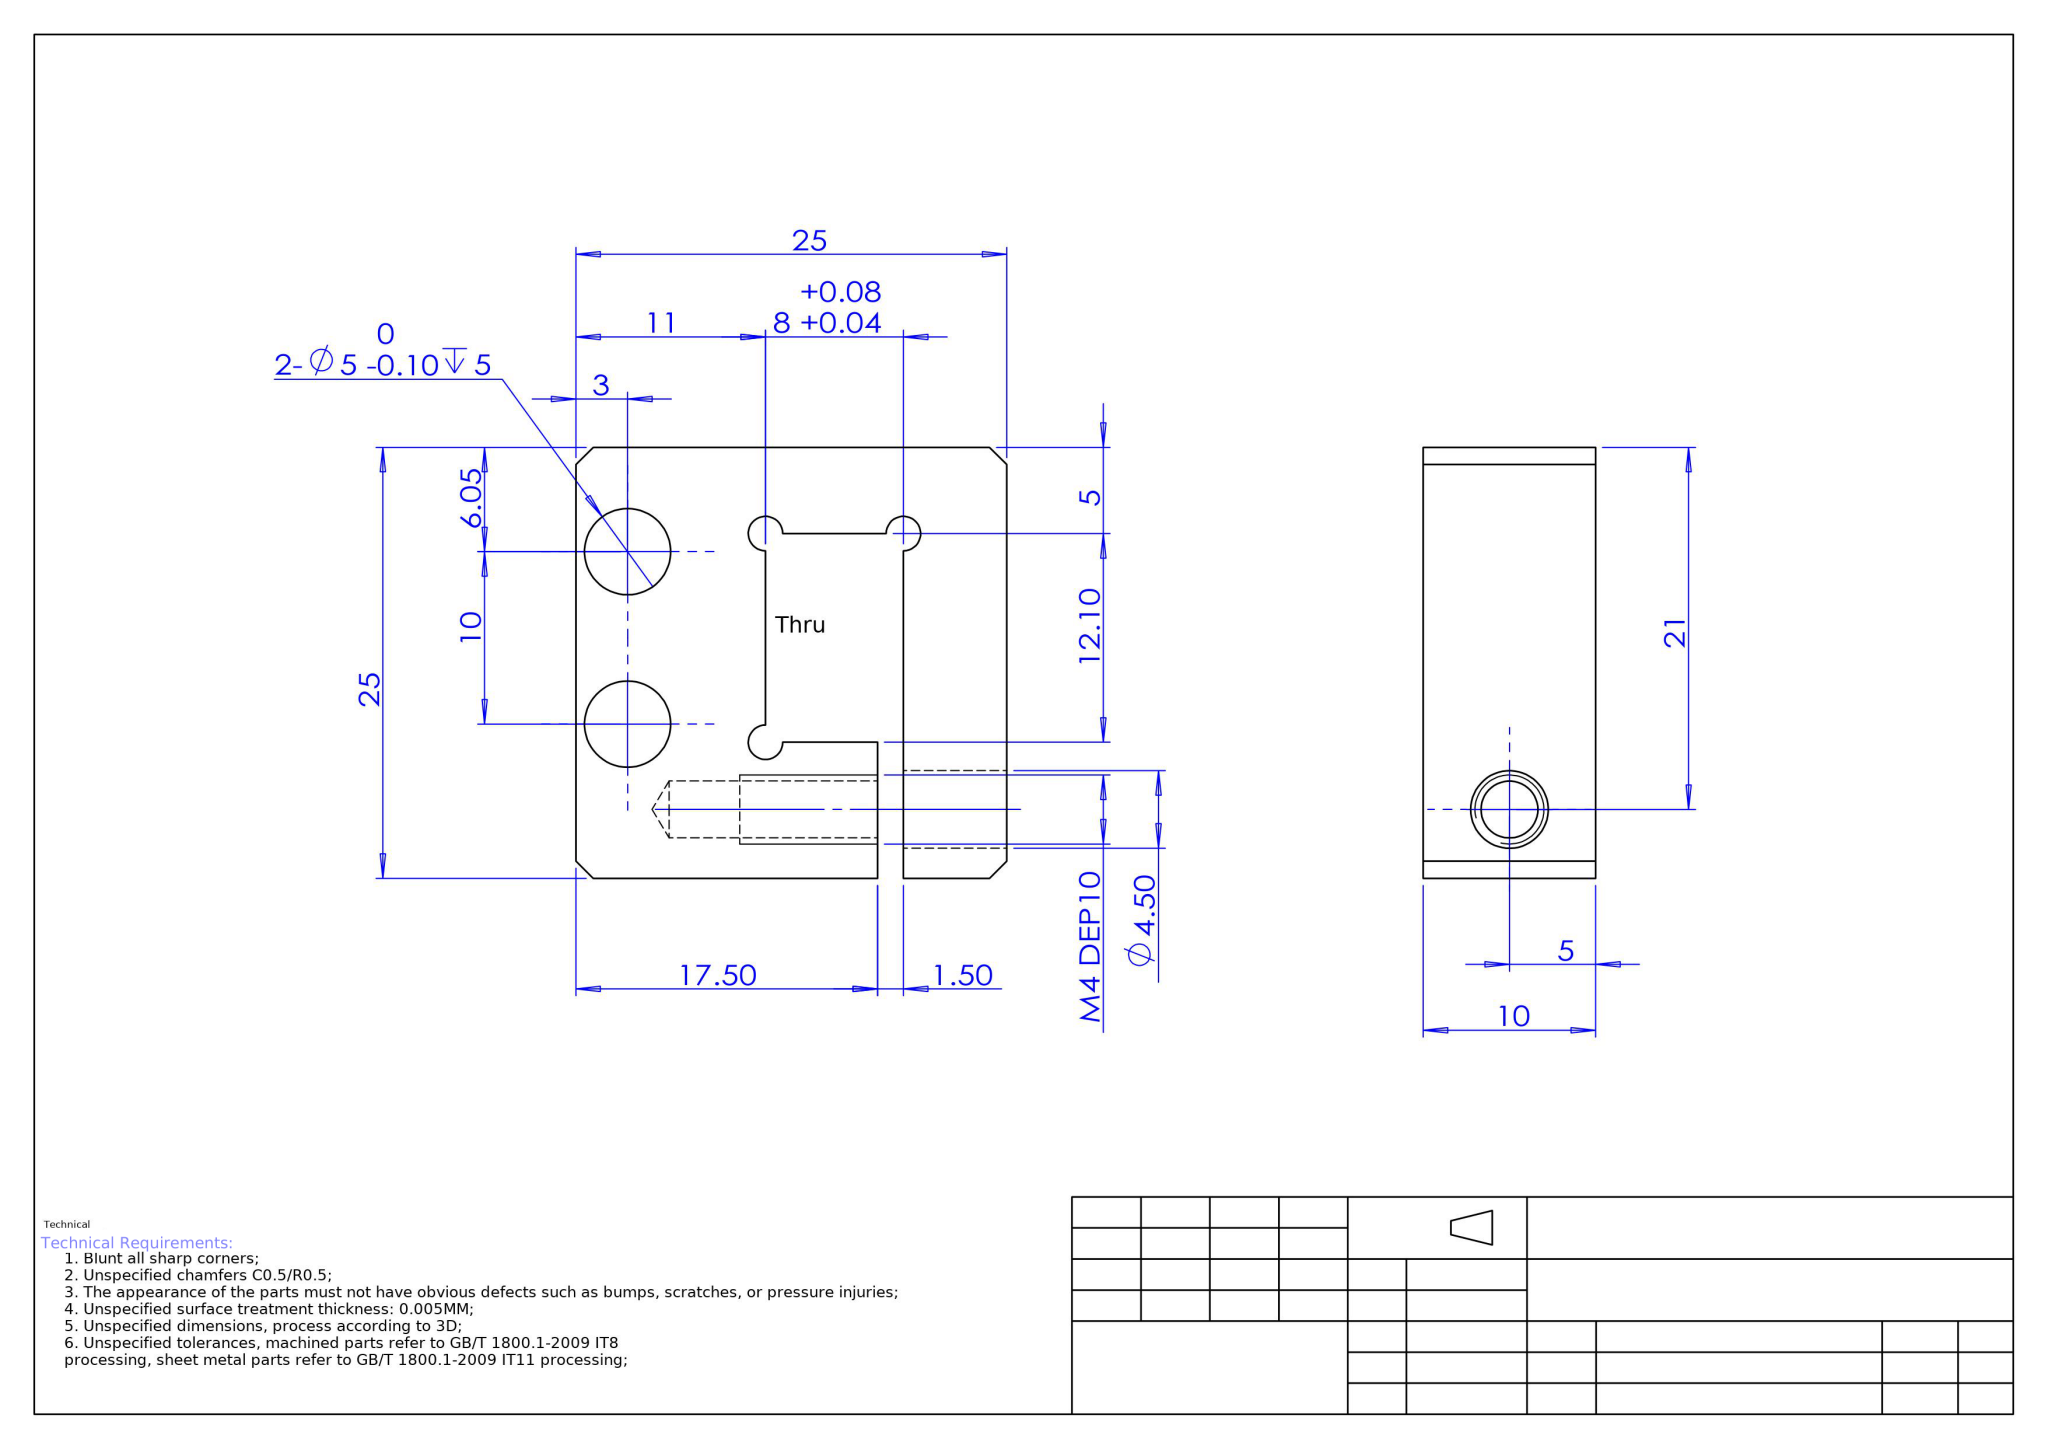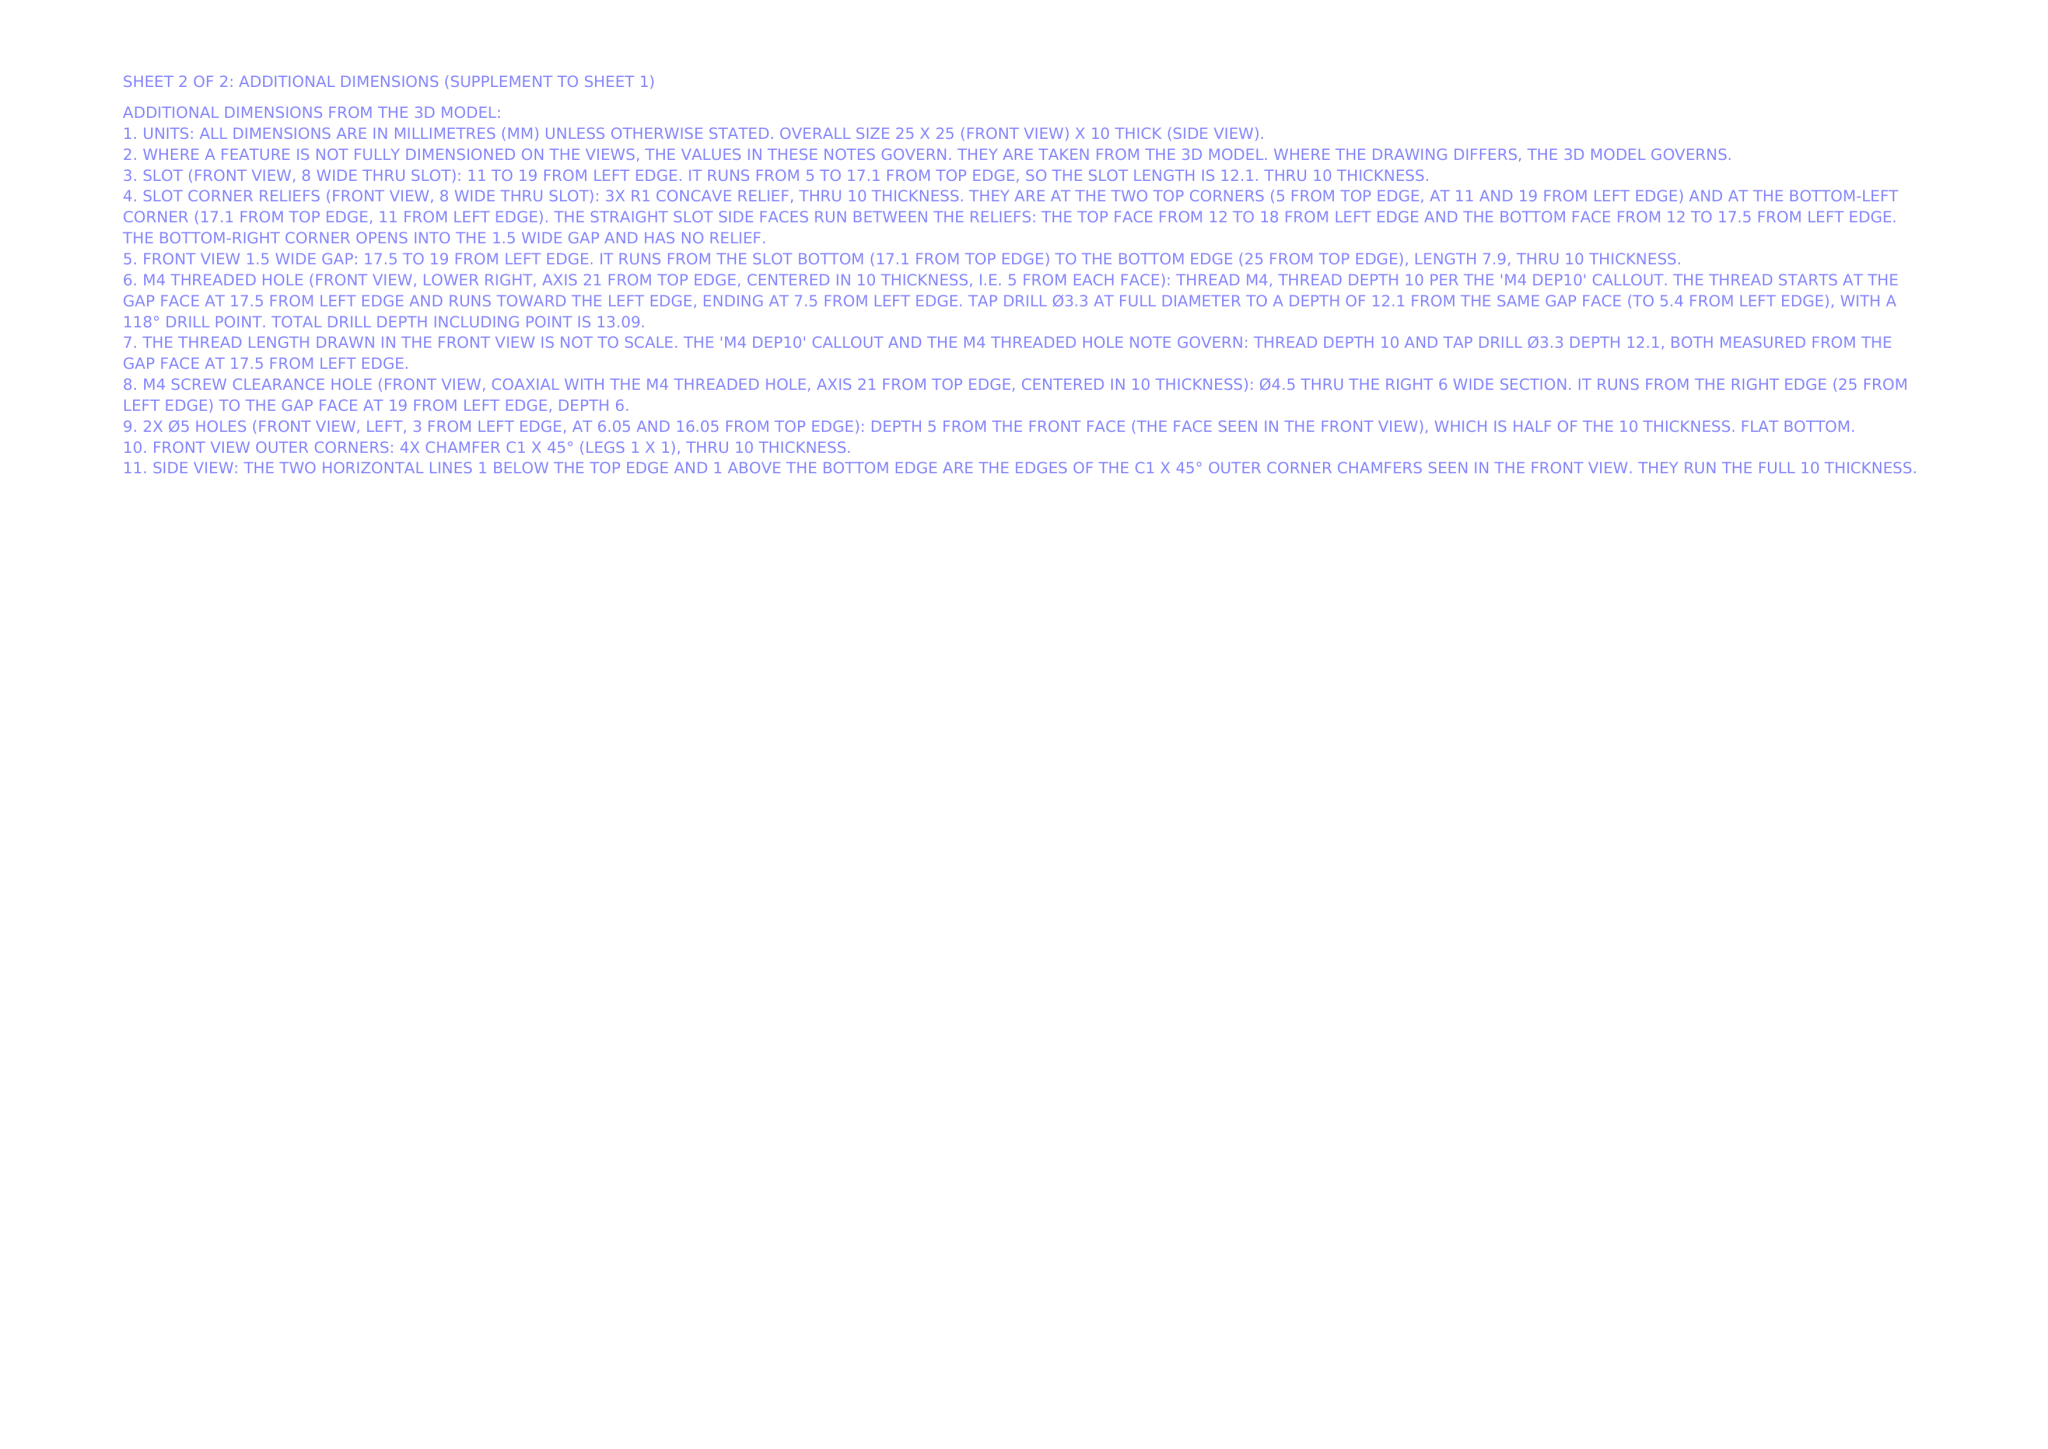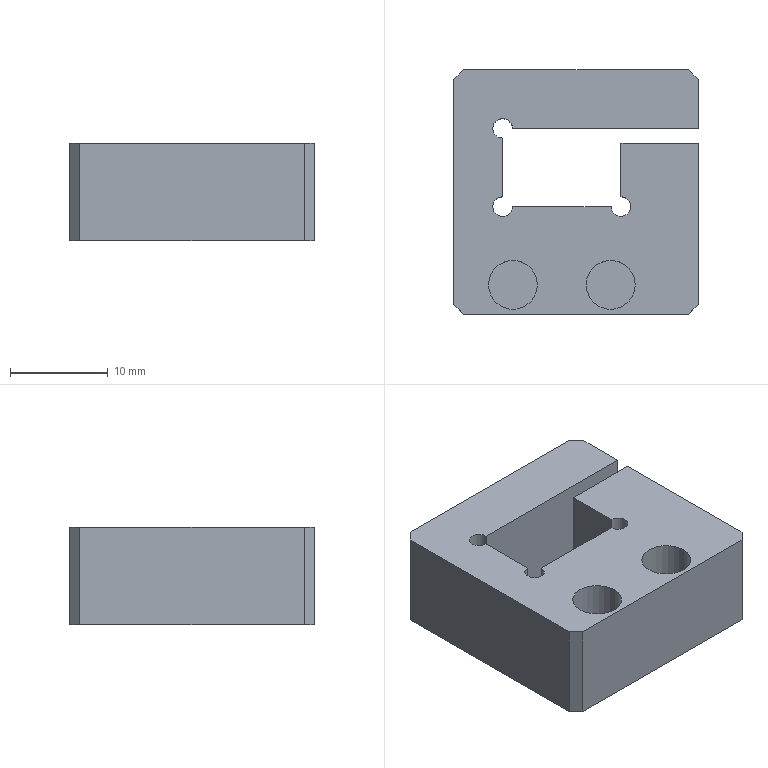Part | NX | mm | 1 solid | 33 faces | box 25 x 25 x 10 mm | volume 4675 mm3 | plane 18 | cylinder 13 | cone 2 | commonest cylinder face diameters 2 x5 5 x4 3.3 x2 4.5 x2